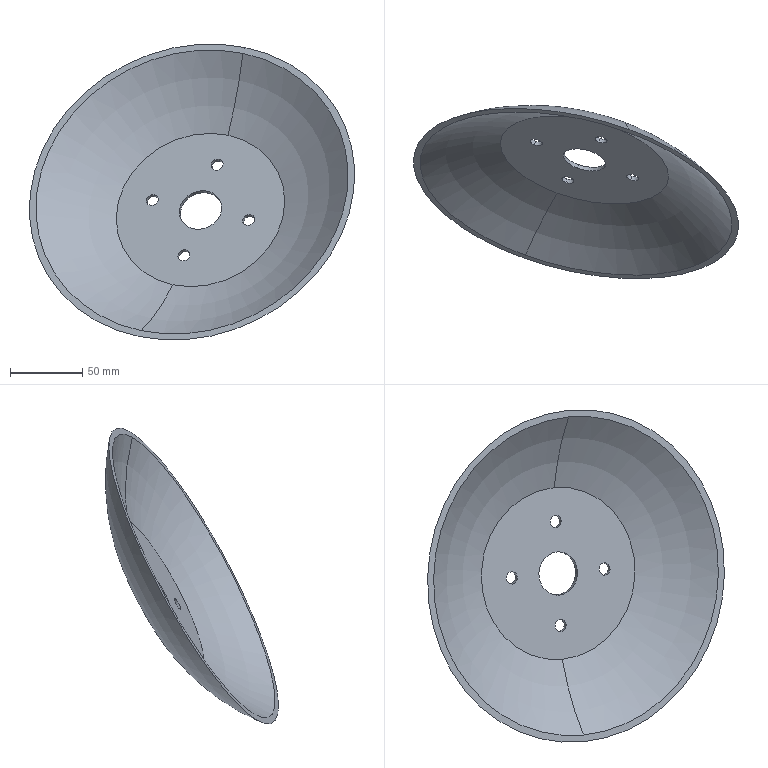Component | SolidWorks | ScribingMechanismAssembly-1_AttachedSoilDiskAssembly-1_AttachedSoilDisk-1 | 1 solid | 17 faces | box 224.52 x 119.34 x 204.2 mm | volume 130350 mm3 | cylinder 10 | torus 4 | plane 3 | commonest cylinder face diameters 8.5 x8 30 x2
STEP:
#1=CARTESIAN_POINT('',(-4.238,3.691,34.243));
#2=VERTEX_POINT('',#1);
#3=CARTESIAN_POINT('',(-4.344,3.562,33.953));
#4=VERTEX_POINT('',#3);
#5=CARTESIAN_POINT('',(-4.291,3.626,34.098));
#6=DIRECTION('',(-0.2171,-0.8609,0.4602));
#7=DIRECTION('',(-0.3178,-0.3834,-0.8672));
#8=AXIS2_PLACEMENT_3D('',#5,#6,#7);
#9=CIRCLE('',#8,0.1673);
#10=EDGE_CURVE('',#2,#4,#9,.T.);
#11=ORIENTED_EDGE('',*,*,#10,.T.);
#12=CARTESIAN_POINT('',(-4.318,3.664,33.899));
#13=VERTEX_POINT('',#12);
#14=CARTESIAN_POINT('',(-4.404,3.325,34.08));
#15=DIRECTION('',(0.2171,0.8609,-0.4602));
#16=VECTOR('',#15,39.37);
#17=LINE('',#14,#16);
#18=EDGE_CURVE('',#4,#13,#17,.T.);
#19=ORIENTED_EDGE('',*,*,#18,.T.);
#20=CARTESIAN_POINT('',(-4.212,3.792,34.189));
#21=VERTEX_POINT('',#20);
#22=CARTESIAN_POINT('',(-4.265,3.728,34.044));
#23=DIRECTION('',(0.2171,0.8609,-0.4602));
#24=DIRECTION('',(-0.923,0.3345,0.1904));
#25=AXIS2_PLACEMENT_3D('',#22,#23,#24);
#26=CIRCLE('',#25,0.1673);
#27=EDGE_CURVE('',#13,#21,#26,.T.);
#28=ORIENTED_EDGE('',*,*,#27,.T.);
#29=CARTESIAN_POINT('',(-4.298,3.453,34.37));
#30=DIRECTION('',(0.2171,0.8609,-0.4602));
#31=VECTOR('',#30,39.37);
#32=LINE('',#29,#31);
#33=EDGE_CURVE('',#2,#21,#32,.T.);
#34=ORIENTED_EDGE('',*,*,#33,.F.);
#35=EDGE_LOOP('',(#11,#19,#28,#34));
#36=FACE_OUTER_BOUND('',#35,.T.);
#37=CARTESIAN_POINT('',(-4.351,3.389,34.225));
#38=DIRECTION('',(0.2171,0.8609,-0.4602));
#39=DIRECTION('',(0.3178,0.3834,0.8672));
#40=AXIS2_PLACEMENT_3D('',#37,#38,#39);
#41=CYLINDRICAL_SURFACE('',#40,0.1673);
#42=ADVANCED_FACE('',(#36),#41,.F.);
#43=CARTESIAN_POINT('',(-3.38,2.673,32.744));
#44=VERTEX_POINT('',#43);
#45=CARTESIAN_POINT('',(-3.486,2.545,32.454));
#46=VERTEX_POINT('',#45);
#47=CARTESIAN_POINT('',(-3.433,2.609,32.599));
#48=DIRECTION('',(-0.2171,-0.8609,0.4602));
#49=DIRECTION('',(-0.3178,-0.3834,-0.8672));
#50=AXIS2_PLACEMENT_3D('',#47,#48,#49);
#51=CIRCLE('',#50,0.1673);
#52=EDGE_CURVE('',#44,#46,#51,.T.);
#53=ORIENTED_EDGE('',*,*,#52,.T.);
#54=CARTESIAN_POINT('',(-3.461,2.646,32.4));
#55=VERTEX_POINT('',#54);
#56=CARTESIAN_POINT('',(-3.546,2.308,32.581));
#57=DIRECTION('',(0.2171,0.8609,-0.4602));
#58=VECTOR('',#57,39.37);
#59=LINE('',#56,#58);
#60=EDGE_CURVE('',#46,#55,#59,.T.);
#61=ORIENTED_EDGE('',*,*,#60,.T.);
#62=CARTESIAN_POINT('',(-3.354,2.775,32.69));
#63=VERTEX_POINT('',#62);
#64=CARTESIAN_POINT('',(-3.408,2.711,32.545));
#65=DIRECTION('',(0.2171,0.8609,-0.4602));
#66=DIRECTION('',(-0.3178,-0.3834,-0.8672));
#67=AXIS2_PLACEMENT_3D('',#64,#65,#66);
#68=CIRCLE('',#67,0.1673);
#69=EDGE_CURVE('',#55,#63,#68,.T.);
#70=ORIENTED_EDGE('',*,*,#69,.T.);
#71=CARTESIAN_POINT('',(-3.44,2.436,32.871));
#72=DIRECTION('',(0.2171,0.8609,-0.4602));
#73=VECTOR('',#72,39.37);
#74=LINE('',#71,#73);
#75=EDGE_CURVE('',#44,#63,#74,.T.);
#76=ORIENTED_EDGE('',*,*,#75,.F.);
#77=EDGE_LOOP('',(#53,#61,#70,#76));
#78=FACE_OUTER_BOUND('',#77,.T.);
#79=CARTESIAN_POINT('',(-3.493,2.372,32.726));
#80=DIRECTION('',(0.2171,0.8609,-0.4602));
#81=DIRECTION('',(0.3178,0.3834,0.8672));
#82=AXIS2_PLACEMENT_3D('',#79,#80,#81);
#83=CYLINDRICAL_SURFACE('',#82,0.1673);
#84=ADVANCED_FACE('',(#78),#83,.F.);
#85=CARTESIAN_POINT('',(-1.621,2.742,33.704));
#86=VERTEX_POINT('',#85);
#87=CARTESIAN_POINT('',(-1.728,2.614,33.413));
#88=VERTEX_POINT('',#87);
#89=CARTESIAN_POINT('',(-1.675,2.678,33.558));
#90=DIRECTION('',(-0.2171,-0.8609,0.4602));
#91=DIRECTION('',(-0.3178,-0.3834,-0.8672));
#92=AXIS2_PLACEMENT_3D('',#89,#90,#91);
#93=CIRCLE('',#92,0.1673);
#94=EDGE_CURVE('',#86,#88,#93,.T.);
#95=ORIENTED_EDGE('',*,*,#94,.T.);
#96=CARTESIAN_POINT('',(-1.702,2.716,33.359));
#97=VERTEX_POINT('',#96);
#98=CARTESIAN_POINT('',(-1.788,2.377,33.54));
#99=DIRECTION('',(0.2171,0.8609,-0.4602));
#100=VECTOR('',#99,39.37);
#101=LINE('',#98,#100);
#102=EDGE_CURVE('',#88,#97,#101,.T.);
#103=ORIENTED_EDGE('',*,*,#102,.T.);
#104=CARTESIAN_POINT('',(-1.596,2.844,33.649));
#105=VERTEX_POINT('',#104);
#106=CARTESIAN_POINT('',(-1.649,2.78,33.504));
#107=DIRECTION('',(0.2171,0.8609,-0.4602));
#108=DIRECTION('',(0.923,-0.3345,-0.1904));
#109=AXIS2_PLACEMENT_3D('',#106,#107,#108);
#110=CIRCLE('',#109,0.1673);
#111=EDGE_CURVE('',#97,#105,#110,.T.);
#112=ORIENTED_EDGE('',*,*,#111,.T.);
#113=CARTESIAN_POINT('',(-1.681,2.505,33.83));
#114=DIRECTION('',(0.2171,0.8609,-0.4602));
#115=VECTOR('',#114,39.37);
#116=LINE('',#113,#115);
#117=EDGE_CURVE('',#86,#105,#116,.T.);
#118=ORIENTED_EDGE('',*,*,#117,.F.);
#119=EDGE_LOOP('',(#95,#103,#112,#118));
#120=FACE_OUTER_BOUND('',#119,.T.);
#121=CARTESIAN_POINT('',(-1.734,2.441,33.685));
#122=DIRECTION('',(0.2171,0.8609,-0.4602));
#123=DIRECTION('',(0.3178,0.3834,0.8672));
#124=AXIS2_PLACEMENT_3D('',#121,#122,#123);
#125=CYLINDRICAL_SURFACE('',#124,0.1673);
#126=ADVANCED_FACE('',(#120),#125,.F.);
#127=CARTESIAN_POINT('',(-2.479,3.76,35.202));
#128=VERTEX_POINT('',#127);
#129=CARTESIAN_POINT('',(-2.585,3.632,34.912));
#130=VERTEX_POINT('',#129);
#131=CARTESIAN_POINT('',(-2.532,3.696,35.057));
#132=DIRECTION('',(-0.2171,-0.8609,0.4602));
#133=DIRECTION('',(-0.3178,-0.3834,-0.8672));
#134=AXIS2_PLACEMENT_3D('',#131,#132,#133);
#135=CIRCLE('',#134,0.1673);
#136=EDGE_CURVE('',#128,#130,#135,.T.);
#137=ORIENTED_EDGE('',*,*,#136,.T.);
#138=CARTESIAN_POINT('',(-2.56,3.733,34.858));
#139=VERTEX_POINT('',#138);
#140=CARTESIAN_POINT('',(-2.645,3.394,35.039));
#141=DIRECTION('',(0.2171,0.8609,-0.4602));
#142=VECTOR('',#141,39.37);
#143=LINE('',#140,#142);
#144=EDGE_CURVE('',#130,#139,#143,.T.);
#145=ORIENTED_EDGE('',*,*,#144,.T.);
#146=CARTESIAN_POINT('',(-2.453,3.862,35.148));
#147=VERTEX_POINT('',#146);
#148=CARTESIAN_POINT('',(-2.507,3.797,35.003));
#149=DIRECTION('',(0.2171,0.8609,-0.4602));
#150=DIRECTION('',(0.3178,0.3834,0.8672));
#151=AXIS2_PLACEMENT_3D('',#148,#149,#150);
#152=CIRCLE('',#151,0.1673);
#153=EDGE_CURVE('',#139,#147,#152,.T.);
#154=ORIENTED_EDGE('',*,*,#153,.T.);
#155=CARTESIAN_POINT('',(-2.539,3.523,35.329));
#156=DIRECTION('',(0.2171,0.8609,-0.4602));
#157=VECTOR('',#156,39.37);
#158=LINE('',#155,#157);
#159=EDGE_CURVE('',#128,#147,#158,.T.);
#160=ORIENTED_EDGE('',*,*,#159,.F.);
#161=EDGE_LOOP('',(#137,#145,#154,#160));
#162=FACE_OUTER_BOUND('',#161,.T.);
#163=CARTESIAN_POINT('',(-2.592,3.458,35.184));
#164=DIRECTION('',(0.2171,0.8609,-0.4602));
#165=DIRECTION('',(0.3178,0.3834,0.8672));
#166=AXIS2_PLACEMENT_3D('',#163,#164,#165);
#167=CYLINDRICAL_SURFACE('',#166,0.1673);
#168=ADVANCED_FACE('',(#162),#167,.F.);
#169=CARTESIAN_POINT('',(-2.795,3.379,34.34));
#170=VERTEX_POINT('',#169);
#171=CARTESIAN_POINT('',(-3.17,2.926,33.316));
#172=VERTEX_POINT('',#171);
#173=CARTESIAN_POINT('',(-2.983,3.152,33.828));
#174=DIRECTION('',(-0.2171,-0.8609,0.4602));
#175=DIRECTION('',(-0.3178,-0.3834,-0.8672));
#176=AXIS2_PLACEMENT_3D('',#173,#174,#175);
#177=CIRCLE('',#176,0.5906);
#178=EDGE_CURVE('',#170,#172,#177,.T.);
#179=ORIENTED_EDGE('',*,*,#178,.T.);
#180=CARTESIAN_POINT('',(-3.145,3.028,33.262));
#181=VERTEX_POINT('',#180);
#182=CARTESIAN_POINT('',(-3.23,2.689,33.443));
#183=DIRECTION('',(0.2171,0.8609,-0.4602));
#184=VECTOR('',#183,39.37);
#185=LINE('',#182,#184);
#186=EDGE_CURVE('',#172,#181,#185,.T.);
#187=ORIENTED_EDGE('',*,*,#186,.T.);
#188=CARTESIAN_POINT('',(-2.769,3.48,34.286));
#189=VERTEX_POINT('',#188);
#190=CARTESIAN_POINT('',(-2.957,3.254,33.774));
#191=DIRECTION('',(0.2171,0.8609,-0.4602));
#192=DIRECTION('',(0.3178,0.3834,0.8672));
#193=AXIS2_PLACEMENT_3D('',#190,#191,#192);
#194=CIRCLE('',#193,0.5906);
#195=EDGE_CURVE('',#181,#189,#194,.T.);
#196=ORIENTED_EDGE('',*,*,#195,.T.);
#197=CARTESIAN_POINT('',(-2.855,3.141,34.467));
#198=DIRECTION('',(0.2171,0.8609,-0.4602));
#199=VECTOR('',#198,39.37);
#200=LINE('',#197,#199);
#201=EDGE_CURVE('',#170,#189,#200,.T.);
#202=ORIENTED_EDGE('',*,*,#201,.F.);
#203=EDGE_LOOP('',(#179,#187,#196,#202));
#204=FACE_OUTER_BOUND('',#203,.T.);
#205=CARTESIAN_POINT('',(-3.043,2.915,33.955));
#206=DIRECTION('',(0.2171,0.8609,-0.4602));
#207=DIRECTION('',(0.3178,0.3834,0.8672));
#208=AXIS2_PLACEMENT_3D('',#205,#206,#207);
#209=CYLINDRICAL_SURFACE('',#208,0.5906);
#210=ADVANCED_FACE('',(#204),#209,.F.);
#211=CARTESIAN_POINT('',(-4.594,0.5718,30.551));
#212=VERTEX_POINT('',#211);
#213=CARTESIAN_POINT('',(-1.833,3.903,38.084));
#214=VERTEX_POINT('',#213);
#215=CARTESIAN_POINT('',(-3.213,2.237,34.317));
#216=DIRECTION('',(0.2171,0.8609,-0.4602));
#217=DIRECTION('',(0.3178,0.3834,0.8672));
#218=AXIS2_PLACEMENT_3D('',#215,#216,#217);
#219=CIRCLE('',#218,4.344);
#220=EDGE_CURVE('',#212,#214,#219,.T.);
#221=ORIENTED_EDGE('',*,*,#220,.F.);
#222=CARTESIAN_POINT('',(-3.728,2.253,31.795));
#223=VERTEX_POINT('',#222);
#224=CARTESIAN_POINT('',(-4.402,-1.88,35.79));
#225=DIRECTION('',(0.923,-0.3345,-0.1904));
#226=DIRECTION('',(0.3407,0.9402,0.));
#227=AXIS2_PLACEMENT_3D('',#224,#225,#226);
#228=CIRCLE('',#227,5.787);
#229=EDGE_CURVE('',#212,#223,#228,.T.);
#230=ORIENTED_EDGE('',*,*,#229,.T.);
#231=CARTESIAN_POINT('',(-2.237,4.051,35.862));
#232=VERTEX_POINT('',#231);
#233=CARTESIAN_POINT('',(-2.983,3.152,33.828));
#234=DIRECTION('',(0.2171,0.8609,-0.4602));
#235=DIRECTION('',(0.3178,0.3834,0.8672));
#236=AXIS2_PLACEMENT_3D('',#233,#234,#235);
#237=CIRCLE('',#236,2.345);
#238=EDGE_CURVE('',#223,#232,#237,.T.);
#239=ORIENTED_EDGE('',*,*,#238,.T.);
#240=CARTESIAN_POINT('',(-3.97,-1.359,36.968));
#241=DIRECTION('',(-0.923,0.3345,0.1904));
#242=DIRECTION('',(-0.3407,-0.9402,0.));
#243=AXIS2_PLACEMENT_3D('',#240,#241,#242);
#244=CIRCLE('',#243,5.787);
#245=EDGE_CURVE('',#214,#232,#244,.T.);
#246=ORIENTED_EDGE('',*,*,#245,.F.);
#247=EDGE_LOOP('',(#221,#230,#239,#246));
#248=FACE_OUTER_BOUND('',#247,.T.);
#249=CARTESIAN_POINT('',(-4.186,-1.619,36.379));
#250=DIRECTION('',(0.2171,0.8609,-0.4602));
#251=DIRECTION('',(0.3178,0.3834,0.8672));
#252=AXIS2_PLACEMENT_3D('',#249,#250,#251);
#253=TOROIDAL_SURFACE('',#252,0.6794,5.787);
#254=ADVANCED_FACE('',(#248),#253,.F.);
#255=CARTESIAN_POINT('',(-1.775,3.973,38.244));
#256=VERTEX_POINT('',#255);
#257=CARTESIAN_POINT('',(-4.652,0.5014,30.391));
#258=VERTEX_POINT('',#257);
#259=CARTESIAN_POINT('',(-3.213,2.237,34.317));
#260=DIRECTION('',(0.2171,0.8609,-0.4602));
#261=DIRECTION('',(0.3178,0.3834,0.8672));
#262=AXIS2_PLACEMENT_3D('',#259,#260,#261);
#263=CIRCLE('',#262,4.528);
#264=EDGE_CURVE('',#256,#258,#263,.T.);
#265=ORIENTED_EDGE('',*,*,#264,.T.);
#266=CARTESIAN_POINT('',(-3.708,2.348,31.725));
#267=VERTEX_POINT('',#266);
#268=CARTESIAN_POINT('',(-4.402,-1.88,35.79));
#269=DIRECTION('',(0.923,-0.3345,-0.1904));
#270=DIRECTION('',(0.3407,0.9402,0.));
#271=AXIS2_PLACEMENT_3D('',#268,#269,#270);
#272=CIRCLE('',#271,5.906);
#273=EDGE_CURVE('',#258,#267,#272,.T.);
#274=ORIENTED_EDGE('',*,*,#273,.T.);
#275=CARTESIAN_POINT('',(-2.206,4.16,35.822));
#276=VERTEX_POINT('',#275);
#277=CARTESIAN_POINT('',(-2.957,3.254,33.774));
#278=DIRECTION('',(0.2171,0.8609,-0.4602));
#279=DIRECTION('',(0.3178,0.3834,0.8672));
#280=AXIS2_PLACEMENT_3D('',#277,#278,#279);
#281=CIRCLE('',#280,2.362);
#282=EDGE_CURVE('',#276,#267,#281,.T.);
#283=ORIENTED_EDGE('',*,*,#282,.F.);
#284=CARTESIAN_POINT('',(-3.97,-1.359,36.968));
#285=DIRECTION('',(-0.923,0.3345,0.1904));
#286=DIRECTION('',(-0.3407,-0.9402,0.));
#287=AXIS2_PLACEMENT_3D('',#284,#285,#286);
#288=CIRCLE('',#287,5.906);
#289=EDGE_CURVE('',#256,#276,#288,.T.);
#290=ORIENTED_EDGE('',*,*,#289,.F.);
#291=EDGE_LOOP('',(#265,#274,#283,#290));
#292=FACE_OUTER_BOUND('',#291,.T.);
#293=CARTESIAN_POINT('',(-4.186,-1.619,36.379));
#294=DIRECTION('',(0.2171,0.8609,-0.4602));
#295=DIRECTION('',(0.3178,0.3834,0.8672));
#296=AXIS2_PLACEMENT_3D('',#293,#294,#295);
#297=TOROIDAL_SURFACE('',#296,0.6794,5.906);
#298=ADVANCED_FACE('',(#292),#297,.T.);
#299=ORIENTED_EDGE('',*,*,#273,.F.);
#300=CARTESIAN_POINT('',(-3.213,2.237,34.317));
#301=DIRECTION('',(0.2171,0.8609,-0.4602));
#302=DIRECTION('',(0.3178,0.3834,0.8672));
#303=AXIS2_PLACEMENT_3D('',#300,#301,#302);
#304=CIRCLE('',#303,4.528);
#305=EDGE_CURVE('',#258,#256,#304,.T.);
#306=ORIENTED_EDGE('',*,*,#305,.T.);
#307=ORIENTED_EDGE('',*,*,#289,.T.);
#308=CARTESIAN_POINT('',(-2.957,3.254,33.774));
#309=DIRECTION('',(0.2171,0.8609,-0.4602));
#310=DIRECTION('',(0.3178,0.3834,0.8672));
#311=AXIS2_PLACEMENT_3D('',#308,#309,#310);
#312=CIRCLE('',#311,2.362);
#313=EDGE_CURVE('',#267,#276,#312,.T.);
#314=ORIENTED_EDGE('',*,*,#313,.F.);
#315=EDGE_LOOP('',(#299,#306,#307,#314));
#316=FACE_OUTER_BOUND('',#315,.T.);
#317=CARTESIAN_POINT('',(-4.186,-1.619,36.379));
#318=DIRECTION('',(0.2171,0.8609,-0.4602));
#319=DIRECTION('',(0.3178,0.3834,0.8672));
#320=AXIS2_PLACEMENT_3D('',#317,#318,#319);
#321=TOROIDAL_SURFACE('',#320,0.6794,5.906);
#322=ADVANCED_FACE('',(#316),#321,.T.);
#323=CARTESIAN_POINT('',(-4.265,3.728,34.044));
#324=DIRECTION('',(0.2171,0.8609,-0.4602));
#325=DIRECTION('',(-0.923,0.3345,0.1904));
#326=AXIS2_PLACEMENT_3D('',#323,#324,#325);
#327=CIRCLE('',#326,0.1673);
#328=EDGE_CURVE('',#21,#13,#327,.T.);
#329=ORIENTED_EDGE('',*,*,#328,.F.);
#330=ORIENTED_EDGE('',*,*,#27,.F.);
#331=EDGE_LOOP('',(#329,#330));
#332=FACE_BOUND('',#331,.T.);
#333=CARTESIAN_POINT('',(-3.408,2.711,32.545));
#334=DIRECTION('',(0.2171,0.8609,-0.4602));
#335=DIRECTION('',(-0.3178,-0.3834,-0.8672));
#336=AXIS2_PLACEMENT_3D('',#333,#334,#335);
#337=CIRCLE('',#336,0.1673);
#338=EDGE_CURVE('',#63,#55,#337,.T.);
#339=ORIENTED_EDGE('',*,*,#338,.F.);
#340=ORIENTED_EDGE('',*,*,#69,.F.);
#341=EDGE_LOOP('',(#339,#340));
#342=FACE_BOUND('',#341,.T.);
#343=CARTESIAN_POINT('',(-1.649,2.78,33.504));
#344=DIRECTION('',(0.2171,0.8609,-0.4602));
#345=DIRECTION('',(0.923,-0.3345,-0.1904));
#346=AXIS2_PLACEMENT_3D('',#343,#344,#345);
#347=CIRCLE('',#346,0.1673);
#348=EDGE_CURVE('',#105,#97,#347,.T.);
#349=ORIENTED_EDGE('',*,*,#348,.F.);
#350=ORIENTED_EDGE('',*,*,#111,.F.);
#351=EDGE_LOOP('',(#349,#350));
#352=FACE_BOUND('',#351,.T.);
#353=CARTESIAN_POINT('',(-2.507,3.797,35.003));
#354=DIRECTION('',(0.2171,0.8609,-0.4602));
#355=DIRECTION('',(0.3178,0.3834,0.8672));
#356=AXIS2_PLACEMENT_3D('',#353,#354,#355);
#357=CIRCLE('',#356,0.1673);
#358=EDGE_CURVE('',#147,#139,#357,.T.);
#359=ORIENTED_EDGE('',*,*,#358,.F.);
#360=ORIENTED_EDGE('',*,*,#153,.F.);
#361=EDGE_LOOP('',(#359,#360));
#362=FACE_BOUND('',#361,.T.);
#363=CARTESIAN_POINT('',(-2.957,3.254,33.774));
#364=DIRECTION('',(0.2171,0.8609,-0.4602));
#365=DIRECTION('',(0.3178,0.3834,0.8672));
#366=AXIS2_PLACEMENT_3D('',#363,#364,#365);
#367=CIRCLE('',#366,0.5906);
#368=EDGE_CURVE('',#189,#181,#367,.T.);
#369=ORIENTED_EDGE('',*,*,#368,.F.);
#370=ORIENTED_EDGE('',*,*,#195,.F.);
#371=EDGE_LOOP('',(#369,#370));
#372=FACE_BOUND('',#371,.T.);
#373=ORIENTED_EDGE('',*,*,#282,.T.);
#374=ORIENTED_EDGE('',*,*,#313,.T.);
#375=EDGE_LOOP('',(#373,#374));
#376=FACE_OUTER_BOUND('',#375,.T.);
#377=CARTESIAN_POINT('',(-2.206,4.16,35.822));
#378=DIRECTION('',(0.2171,0.8609,-0.4602));
#379=DIRECTION('',(0.3178,0.3834,0.8672));
#380=AXIS2_PLACEMENT_3D('',#377,#378,#379);
#381=PLANE('',#380);
#382=ADVANCED_FACE('',(#332,#342,#352,#362,#372,#376),#381,.T.);
#383=ORIENTED_EDGE('',*,*,#10,.F.);
#384=CARTESIAN_POINT('',(-4.291,3.626,34.098));
#385=DIRECTION('',(-0.2171,-0.8609,0.4602));
#386=DIRECTION('',(-0.3178,-0.3834,-0.8672));
#387=AXIS2_PLACEMENT_3D('',#384,#385,#386);
#388=CIRCLE('',#387,0.1673);
#389=EDGE_CURVE('',#4,#2,#388,.T.);
#390=ORIENTED_EDGE('',*,*,#389,.F.);
#391=EDGE_LOOP('',(#383,#390));
#392=FACE_BOUND('',#391,.T.);
#393=ORIENTED_EDGE('',*,*,#52,.F.);
#394=CARTESIAN_POINT('',(-3.433,2.609,32.599));
#395=DIRECTION('',(-0.2171,-0.8609,0.4602));
#396=DIRECTION('',(-0.3178,-0.3834,-0.8672));
#397=AXIS2_PLACEMENT_3D('',#394,#395,#396);
#398=CIRCLE('',#397,0.1673);
#399=EDGE_CURVE('',#46,#44,#398,.T.);
#400=ORIENTED_EDGE('',*,*,#399,.F.);
#401=EDGE_LOOP('',(#393,#400));
#402=FACE_BOUND('',#401,.T.);
#403=ORIENTED_EDGE('',*,*,#94,.F.);
#404=CARTESIAN_POINT('',(-1.675,2.678,33.558));
#405=DIRECTION('',(-0.2171,-0.8609,0.4602));
#406=DIRECTION('',(-0.3178,-0.3834,-0.8672));
#407=AXIS2_PLACEMENT_3D('',#404,#405,#406);
#408=CIRCLE('',#407,0.1673);
#409=EDGE_CURVE('',#88,#86,#408,.T.);
#410=ORIENTED_EDGE('',*,*,#409,.F.);
#411=EDGE_LOOP('',(#403,#410));
#412=FACE_BOUND('',#411,.T.);
#413=ORIENTED_EDGE('',*,*,#136,.F.);
#414=CARTESIAN_POINT('',(-2.532,3.696,35.057));
#415=DIRECTION('',(-0.2171,-0.8609,0.4602));
#416=DIRECTION('',(-0.3178,-0.3834,-0.8672));
#417=AXIS2_PLACEMENT_3D('',#414,#415,#416);
#418=CIRCLE('',#417,0.1673);
#419=EDGE_CURVE('',#130,#128,#418,.T.);
#420=ORIENTED_EDGE('',*,*,#419,.F.);
#421=EDGE_LOOP('',(#413,#420));
#422=FACE_BOUND('',#421,.T.);
#423=ORIENTED_EDGE('',*,*,#178,.F.);
#424=CARTESIAN_POINT('',(-2.983,3.152,33.828));
#425=DIRECTION('',(-0.2171,-0.8609,0.4602));
#426=DIRECTION('',(-0.3178,-0.3834,-0.8672));
#427=AXIS2_PLACEMENT_3D('',#424,#425,#426);
#428=CIRCLE('',#427,0.5906);
#429=EDGE_CURVE('',#172,#170,#428,.T.);
#430=ORIENTED_EDGE('',*,*,#429,.F.);
#431=EDGE_LOOP('',(#423,#430));
#432=FACE_BOUND('',#431,.T.);
#433=CARTESIAN_POINT('',(-2.983,3.152,33.828));
#434=DIRECTION('',(0.2171,0.8609,-0.4602));
#435=DIRECTION('',(0.3178,0.3834,0.8672));
#436=AXIS2_PLACEMENT_3D('',#433,#434,#435);
#437=CIRCLE('',#436,2.345);
#438=EDGE_CURVE('',#232,#223,#437,.T.);
#439=ORIENTED_EDGE('',*,*,#438,.F.);
#440=ORIENTED_EDGE('',*,*,#238,.F.);
#441=EDGE_LOOP('',(#439,#440));
#442=FACE_OUTER_BOUND('',#441,.T.);
#443=CARTESIAN_POINT('',(-2.237,4.051,35.862));
#444=DIRECTION('',(-0.2171,-0.8609,0.4602));
#445=DIRECTION('',(-0.3178,-0.3834,-0.8672));
#446=AXIS2_PLACEMENT_3D('',#443,#444,#445);
#447=PLANE('',#446);
#448=ADVANCED_FACE('',(#392,#402,#412,#422,#432,#442),#447,.T.);
#449=ORIENTED_EDGE('',*,*,#229,.F.);
#450=CARTESIAN_POINT('',(-3.213,2.237,34.317));
#451=DIRECTION('',(0.2171,0.8609,-0.4602));
#452=DIRECTION('',(0.3178,0.3834,0.8672));
#453=AXIS2_PLACEMENT_3D('',#450,#451,#452);
#454=CIRCLE('',#453,4.344);
#455=EDGE_CURVE('',#214,#212,#454,.T.);
#456=ORIENTED_EDGE('',*,*,#455,.F.);
#457=ORIENTED_EDGE('',*,*,#245,.T.);
#458=ORIENTED_EDGE('',*,*,#438,.T.);
#459=EDGE_LOOP('',(#449,#456,#457,#458));
#460=FACE_OUTER_BOUND('',#459,.T.);
#461=CARTESIAN_POINT('',(-4.186,-1.619,36.379));
#462=DIRECTION('',(0.2171,0.8609,-0.4602));
#463=DIRECTION('',(0.3178,0.3834,0.8672));
#464=AXIS2_PLACEMENT_3D('',#461,#462,#463);
#465=TOROIDAL_SURFACE('',#464,0.6794,5.787);
#466=ADVANCED_FACE('',(#460),#465,.F.);
#467=ORIENTED_EDGE('',*,*,#455,.T.);
#468=ORIENTED_EDGE('',*,*,#220,.T.);
#469=EDGE_LOOP('',(#467,#468));
#470=FACE_BOUND('',#469,.T.);
#471=ORIENTED_EDGE('',*,*,#264,.F.);
#472=ORIENTED_EDGE('',*,*,#305,.F.);
#473=EDGE_LOOP('',(#471,#472));
#474=FACE_OUTER_BOUND('',#473,.T.);
#475=CARTESIAN_POINT('',(-1.833,3.903,38.084));
#476=DIRECTION('',(-0.2171,-0.8609,0.4602));
#477=DIRECTION('',(-0.3178,-0.3834,-0.8672));
#478=AXIS2_PLACEMENT_3D('',#475,#476,#477);
#479=PLANE('',#478);
#480=ADVANCED_FACE('',(#470,#474),#479,.T.);
#481=ORIENTED_EDGE('',*,*,#186,.F.);
#482=ORIENTED_EDGE('',*,*,#429,.T.);
#483=ORIENTED_EDGE('',*,*,#201,.T.);
#484=ORIENTED_EDGE('',*,*,#368,.T.);
#485=EDGE_LOOP('',(#481,#482,#483,#484));
#486=FACE_OUTER_BOUND('',#485,.T.);
#487=CARTESIAN_POINT('',(-3.043,2.915,33.955));
#488=DIRECTION('',(0.2171,0.8609,-0.4602));
#489=DIRECTION('',(0.3178,0.3834,0.8672));
#490=AXIS2_PLACEMENT_3D('',#487,#488,#489);
#491=CYLINDRICAL_SURFACE('',#490,0.5906);
#492=ADVANCED_FACE('',(#486),#491,.F.);
#493=ORIENTED_EDGE('',*,*,#144,.F.);
#494=ORIENTED_EDGE('',*,*,#419,.T.);
#495=ORIENTED_EDGE('',*,*,#159,.T.);
#496=ORIENTED_EDGE('',*,*,#358,.T.);
#497=EDGE_LOOP('',(#493,#494,#495,#496));
#498=FACE_OUTER_BOUND('',#497,.T.);
#499=CARTESIAN_POINT('',(-2.592,3.458,35.184));
#500=DIRECTION('',(0.2171,0.8609,-0.4602));
#501=DIRECTION('',(0.3178,0.3834,0.8672));
#502=AXIS2_PLACEMENT_3D('',#499,#500,#501);
#503=CYLINDRICAL_SURFACE('',#502,0.1673);
#504=ADVANCED_FACE('',(#498),#503,.F.);
#505=ORIENTED_EDGE('',*,*,#102,.F.);
#506=ORIENTED_EDGE('',*,*,#409,.T.);
#507=ORIENTED_EDGE('',*,*,#117,.T.);
#508=ORIENTED_EDGE('',*,*,#348,.T.);
#509=EDGE_LOOP('',(#505,#506,#507,#508));
#510=FACE_OUTER_BOUND('',#509,.T.);
#511=CARTESIAN_POINT('',(-1.734,2.441,33.685));
#512=DIRECTION('',(0.2171,0.8609,-0.4602));
#513=DIRECTION('',(0.3178,0.3834,0.8672));
#514=AXIS2_PLACEMENT_3D('',#511,#512,#513);
#515=CYLINDRICAL_SURFACE('',#514,0.1673);
#516=ADVANCED_FACE('',(#510),#515,.F.);
#517=ORIENTED_EDGE('',*,*,#60,.F.);
#518=ORIENTED_EDGE('',*,*,#399,.T.);
#519=ORIENTED_EDGE('',*,*,#75,.T.);
#520=ORIENTED_EDGE('',*,*,#338,.T.);
#521=EDGE_LOOP('',(#517,#518,#519,#520));
#522=FACE_OUTER_BOUND('',#521,.T.);
#523=CARTESIAN_POINT('',(-3.493,2.372,32.726));
#524=DIRECTION('',(0.2171,0.8609,-0.4602));
#525=DIRECTION('',(0.3178,0.3834,0.8672));
#526=AXIS2_PLACEMENT_3D('',#523,#524,#525);
#527=CYLINDRICAL_SURFACE('',#526,0.1673);
#528=ADVANCED_FACE('',(#522),#527,.F.);
#529=ORIENTED_EDGE('',*,*,#18,.F.);
#530=ORIENTED_EDGE('',*,*,#389,.T.);
#531=ORIENTED_EDGE('',*,*,#33,.T.);
#532=ORIENTED_EDGE('',*,*,#328,.T.);
#533=EDGE_LOOP('',(#529,#530,#531,#532));
#534=FACE_OUTER_BOUND('',#533,.T.);
#535=CARTESIAN_POINT('',(-4.351,3.389,34.225));
#536=DIRECTION('',(0.2171,0.8609,-0.4602));
#537=DIRECTION('',(0.3178,0.3834,0.8672));
#538=AXIS2_PLACEMENT_3D('',#535,#536,#537);
#539=CYLINDRICAL_SURFACE('',#538,0.1673);
#540=ADVANCED_FACE('',(#534),#539,.F.);
#541=CLOSED_SHELL('',(#42,#84,#126,#168,#210,#254,#298,#322,#382,#448,#466,#480,#492,#504,#516,#528,#540));
#542=MANIFOLD_SOLID_BREP('',#541);
#543=CARTESIAN_POINT('',(0.,0.,0.));
#544=DIRECTION('',(0.,0.,1.));
#545=DIRECTION('',(1.,0.,0.));
#546=AXIS2_PLACEMENT_3D('',#543,#544,#545);
#547=(LENGTH_UNIT()NAMED_UNIT(*)SI_UNIT($,.METRE.));
#548=LENGTH_MEASURE_WITH_UNIT(LENGTH_MEASURE(0.0254),#547);
#549=DIMENSIONAL_EXPONENTS(1.,0.,0.,0.,0.,0.,0.);
#550=(CONVERSION_BASED_UNIT('',#548)LENGTH_UNIT()NAMED_UNIT(#549));
#551=UNCERTAINTY_MEASURE_WITH_UNIT(LENGTH_MEASURE(0.00001),#550,'','');
#552=(NAMED_UNIT(*)PLANE_ANGLE_UNIT()SI_UNIT($,.RADIAN.));
#553=(NAMED_UNIT(*)SI_UNIT($,.STERADIAN.)SOLID_ANGLE_UNIT());
#554=(GEOMETRIC_REPRESENTATION_CONTEXT(3)GLOBAL_UNCERTAINTY_ASSIGNED_CONTEXT((#551))GLOBAL_UNIT_ASSIGNED_CONTEXT((#550,#552,#553))REPRESENTATION_CONTEXT('',''));
#555=ADVANCED_BREP_SHAPE_REPRESENTATION('',(#542,#546),#554);
#556=COLOUR_RGB('',0.7922,0.8196,0.9333);
#557=FILL_AREA_STYLE_COLOUR('',#556);
#558=FILL_AREA_STYLE('',(#557));
#559=SURFACE_STYLE_FILL_AREA(#558);
#560=SURFACE_SIDE_STYLE('',(#559));
#561=SURFACE_STYLE_USAGE(.BOTH.,#560);
#562=PRESENTATION_STYLE_ASSIGNMENT((#561));
#563=STYLED_ITEM('',(#562),#542);
#564=(LENGTH_UNIT()NAMED_UNIT(*)SI_UNIT($,.METRE.));
#565=LENGTH_MEASURE_WITH_UNIT(LENGTH_MEASURE(0.0254),#564);
#566=DIMENSIONAL_EXPONENTS(1.,0.,0.,0.,0.,0.,0.);
#567=(CONVERSION_BASED_UNIT('',#565)LENGTH_UNIT()NAMED_UNIT(#566));
#568=UNCERTAINTY_MEASURE_WITH_UNIT(LENGTH_MEASURE(0.00001),#567,'','');
#569=(NAMED_UNIT(*)PLANE_ANGLE_UNIT()SI_UNIT($,.RADIAN.));
#570=(NAMED_UNIT(*)SI_UNIT($,.STERADIAN.)SOLID_ANGLE_UNIT());
#571=(GEOMETRIC_REPRESENTATION_CONTEXT(3)GLOBAL_UNCERTAINTY_ASSIGNED_CONTEXT((#568))GLOBAL_UNIT_ASSIGNED_CONTEXT((#567,#569,#570))REPRESENTATION_CONTEXT('',''));
#572=MECHANICAL_DESIGN_GEOMETRIC_PRESENTATION_REPRESENTATION('',(#563),#571);
#573=PRESENTATION_LAYER_ASSIGNMENT('','',(#563));